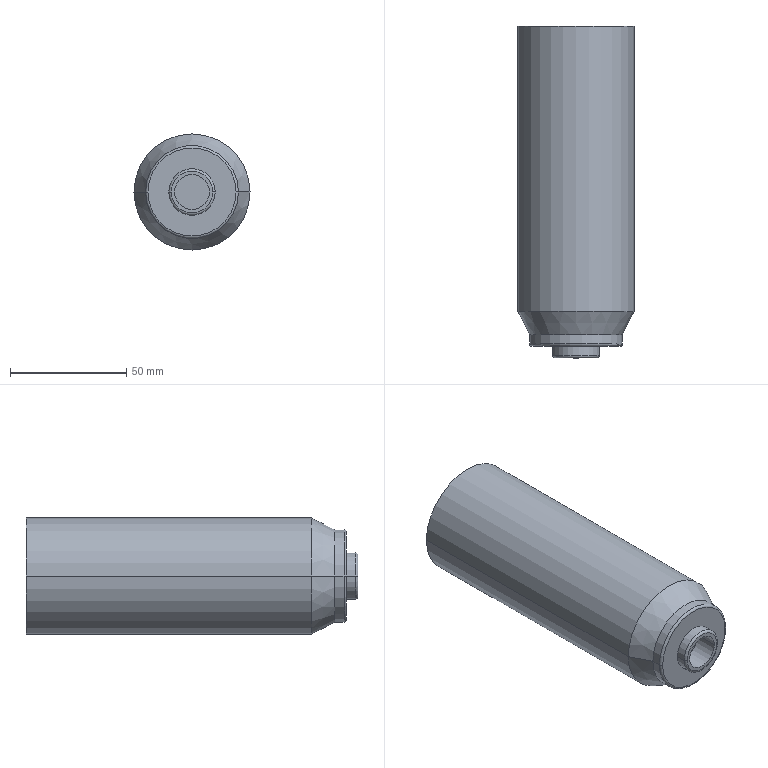Component | SolidWorks | Assembly4.1-1_Ultrasonic.1-1 | 1 solid | 18 faces | box 50 x 143 x 50 mm | volume 263527 mm3 | cylinder 8 | torus 4 | plane 4 | cone 2 | commonest cylinder face diameters 50 x2 40 x2 20 x2 15 x2
build123d program:
from build123d import *


with BuildPart() as part:
    # Sketch1 → Revolve1 (revolve)
    with BuildSketch(Plane.XY, mode=Mode.PRIVATE) as revolve1_sk:
        with BuildLine():
            Line((123, 25), (133, 20))
            Line((133, 20), (137, 20))
            ThreePointArc((137, 20), (137.707, 19.707), (138, 19))
            Line((138, 19), (138, 10))
            Line((138, 10), (142, 10))
            ThreePointArc((142, 10), (142.707, 9.707), (143, 9))
            Line((143, 9), (143, 7.5))
            Line((143, 7.5), (133, 7.5))
            Line((133, 7.5), (133, 0))
            Line((133, 0), (0, 0))
            Line((0, 0), (0, 25))
            Line((0, 25), (123, 25))
        make_face()
    revolve(revolve1_sk.sketch.rotate(Axis((-91.654, 0, 0), (1, 0, 0)), 90), axis=Axis((-91.654, 0, 0), (1, 0, 0)))


solid = part.part

# Placed as in the assembly
solid = solid.moved(Location((0, -101.5, -0.4), (0, 0, -90)))
STEP:
#1=COLOUR_RGB('',0.7922,0.8196,0.9333);
#2=FILL_AREA_STYLE_COLOUR('',#1);
#3=FILL_AREA_STYLE('',(#2));
#4=SURFACE_STYLE_FILL_AREA(#3);
#5=SURFACE_SIDE_STYLE('',(#4));
#6=SURFACE_STYLE_USAGE(.BOTH.,#5);
#7=PRESENTATION_STYLE_ASSIGNMENT((#6));
#8=CARTESIAN_POINT('',(-0.9843,-8.839,-0.01575));
#9=VERTEX_POINT('',#8);
#10=CARTESIAN_POINT('',(0.9843,-8.839,-0.01575));
#11=VERTEX_POINT('',#10);
#12=CARTESIAN_POINT('',(-0.,-8.839,-0.01575));
#13=DIRECTION('',(0.,1.,-0.));
#14=DIRECTION('',(-1.,0.,-0.));
#15=AXIS2_PLACEMENT_3D('',#12,#13,#14);
#16=CIRCLE('',#15,0.9843);
#17=EDGE_CURVE('',#9,#11,#16,.T.);
#18=ORIENTED_EDGE('',*,*,#17,.T.);
#19=CARTESIAN_POINT('',(0.9843,-3.996,-0.01575));
#20=VERTEX_POINT('',#19);
#21=CARTESIAN_POINT('',(0.9843,-0.3877,-0.01575));
#22=DIRECTION('',(0.,1.,-0.));
#23=VECTOR('',#22,39.37);
#24=LINE('',#21,#23);
#25=EDGE_CURVE('',#11,#20,#24,.T.);
#26=ORIENTED_EDGE('',*,*,#25,.T.);
#27=CARTESIAN_POINT('',(-0.9843,-3.996,-0.01575));
#28=VERTEX_POINT('',#27);
#29=CARTESIAN_POINT('',(-0.,-3.996,-0.01575));
#30=DIRECTION('',(0.,1.,-0.));
#31=DIRECTION('',(-1.,0.,-0.));
#32=AXIS2_PLACEMENT_3D('',#29,#30,#31);
#33=CIRCLE('',#32,0.9843);
#34=EDGE_CURVE('',#28,#20,#33,.T.);
#35=ORIENTED_EDGE('',*,*,#34,.F.);
#36=CARTESIAN_POINT('',(-0.9843,-0.3877,-0.01575));
#37=DIRECTION('',(0.,1.,-0.));
#38=VECTOR('',#37,39.37);
#39=LINE('',#36,#38);
#40=EDGE_CURVE('',#9,#28,#39,.T.);
#41=ORIENTED_EDGE('',*,*,#40,.F.);
#42=EDGE_LOOP('',(#18,#26,#35,#41));
#43=FACE_OUTER_BOUND('',#42,.T.);
#44=CARTESIAN_POINT('',(-0.,-0.3877,-0.01575));
#45=DIRECTION('',(0.,1.,-0.));
#46=DIRECTION('',(-1.,0.,-0.));
#47=AXIS2_PLACEMENT_3D('',#44,#45,#46);
#48=CYLINDRICAL_SURFACE('',#47,0.9843);
#49=ADVANCED_FACE('',(#43),#48,.T.);
#50=CARTESIAN_POINT('',(-0.7874,-9.232,-0.01575));
#51=VERTEX_POINT('',#50);
#52=CARTESIAN_POINT('',(0.7874,-9.232,-0.01575));
#53=VERTEX_POINT('',#52);
#54=CARTESIAN_POINT('',(-0.,-9.232,-0.01575));
#55=DIRECTION('',(0.,1.,-0.));
#56=DIRECTION('',(-1.,0.,-0.));
#57=AXIS2_PLACEMENT_3D('',#54,#55,#56);
#58=CIRCLE('',#57,0.7874);
#59=EDGE_CURVE('',#51,#53,#58,.T.);
#60=ORIENTED_EDGE('',*,*,#59,.T.);
#61=CARTESIAN_POINT('',(0.7874,-9.232,-0.01575));
#62=DIRECTION('',(0.4472,0.8944,0.));
#63=VECTOR('',#62,39.37);
#64=LINE('',#61,#63);
#65=EDGE_CURVE('',#53,#11,#64,.T.);
#66=ORIENTED_EDGE('',*,*,#65,.T.);
#67=ORIENTED_EDGE('',*,*,#17,.F.);
#68=CARTESIAN_POINT('',(-0.7874,-9.232,-0.01575));
#69=DIRECTION('',(-0.4472,0.8944,-0.));
#70=VECTOR('',#69,39.37);
#71=LINE('',#68,#70);
#72=EDGE_CURVE('',#51,#9,#71,.T.);
#73=ORIENTED_EDGE('',*,*,#72,.F.);
#74=EDGE_LOOP('',(#60,#66,#67,#73));
#75=FACE_OUTER_BOUND('',#74,.T.);
#76=CARTESIAN_POINT('',(-0.,-9.232,-0.01575));
#77=DIRECTION('',(0.,1.,-0.));
#78=DIRECTION('',(-1.,0.,-0.));
#79=AXIS2_PLACEMENT_3D('',#76,#77,#78);
#80=CONICAL_SURFACE('',#79,0.7874,0.4636);
#81=ADVANCED_FACE('',(#75),#80,.T.);
#82=CARTESIAN_POINT('',(-0.7874,-9.39,-0.01575));
#83=VERTEX_POINT('',#82);
#84=CARTESIAN_POINT('',(0.7874,-9.39,-0.01575));
#85=VERTEX_POINT('',#84);
#86=CARTESIAN_POINT('',(-0.,-9.39,-0.01575));
#87=DIRECTION('',(0.,1.,-0.));
#88=DIRECTION('',(-1.,0.,-0.));
#89=AXIS2_PLACEMENT_3D('',#86,#87,#88);
#90=CIRCLE('',#89,0.7874);
#91=EDGE_CURVE('',#83,#85,#90,.T.);
#92=ORIENTED_EDGE('',*,*,#91,.T.);
#93=CARTESIAN_POINT('',(0.7874,-0.3877,-0.01575));
#94=DIRECTION('',(0.,1.,-0.));
#95=VECTOR('',#94,39.37);
#96=LINE('',#93,#95);
#97=EDGE_CURVE('',#85,#53,#96,.T.);
#98=ORIENTED_EDGE('',*,*,#97,.T.);
#99=ORIENTED_EDGE('',*,*,#59,.F.);
#100=CARTESIAN_POINT('',(-0.7874,-0.3877,-0.01575));
#101=DIRECTION('',(0.,1.,-0.));
#102=VECTOR('',#101,39.37);
#103=LINE('',#100,#102);
#104=EDGE_CURVE('',#83,#51,#103,.T.);
#105=ORIENTED_EDGE('',*,*,#104,.F.);
#106=EDGE_LOOP('',(#92,#98,#99,#105));
#107=FACE_OUTER_BOUND('',#106,.T.);
#108=CARTESIAN_POINT('',(-0.,-0.3877,-0.01575));
#109=DIRECTION('',(0.,1.,-0.));
#110=DIRECTION('',(-1.,0.,-0.));
#111=AXIS2_PLACEMENT_3D('',#108,#109,#110);
#112=CYLINDRICAL_SURFACE('',#111,0.7874);
#113=ADVANCED_FACE('',(#107),#112,.T.);
#114=CARTESIAN_POINT('',(-0.748,-9.429,-0.01575));
#115=VERTEX_POINT('',#114);
#116=CARTESIAN_POINT('',(0.748,-9.429,-0.01575));
#117=VERTEX_POINT('',#116);
#118=CARTESIAN_POINT('',(-0.,-9.429,-0.01575));
#119=DIRECTION('',(0.,1.,-0.));
#120=DIRECTION('',(-1.,0.,-0.));
#121=AXIS2_PLACEMENT_3D('',#118,#119,#120);
#122=CIRCLE('',#121,0.748);
#123=EDGE_CURVE('',#115,#117,#122,.T.);
#124=ORIENTED_EDGE('',*,*,#123,.T.);
#125=CARTESIAN_POINT('',(0.748,-9.39,-0.01575));
#126=DIRECTION('',(-0.,0.,1.));
#127=DIRECTION('',(1.,0.,0.));
#128=AXIS2_PLACEMENT_3D('',#125,#126,#127);
#129=CIRCLE('',#128,0.03937);
#130=EDGE_CURVE('',#117,#85,#129,.T.);
#131=ORIENTED_EDGE('',*,*,#130,.T.);
#132=ORIENTED_EDGE('',*,*,#91,.F.);
#133=CARTESIAN_POINT('',(-0.748,-9.39,-0.01575));
#134=DIRECTION('',(0.,-0.,-1.));
#135=DIRECTION('',(-1.,0.,-0.));
#136=AXIS2_PLACEMENT_3D('',#133,#134,#135);
#137=CIRCLE('',#136,0.03937);
#138=EDGE_CURVE('',#115,#83,#137,.T.);
#139=ORIENTED_EDGE('',*,*,#138,.F.);
#140=EDGE_LOOP('',(#124,#131,#132,#139));
#141=FACE_OUTER_BOUND('',#140,.T.);
#142=CARTESIAN_POINT('',(-0.,-9.39,-0.01575));
#143=DIRECTION('',(0.,1.,-0.));
#144=DIRECTION('',(-1.,0.,-0.));
#145=AXIS2_PLACEMENT_3D('',#142,#143,#144);
#146=TOROIDAL_SURFACE('',#145,0.748,0.03937);
#147=ADVANCED_FACE('',(#141),#146,.T.);
#148=CARTESIAN_POINT('',(-0.3937,-9.587,-0.01575));
#149=VERTEX_POINT('',#148);
#150=CARTESIAN_POINT('',(0.3937,-9.587,-0.01575));
#151=VERTEX_POINT('',#150);
#152=CARTESIAN_POINT('',(-0.,-9.587,-0.01575));
#153=DIRECTION('',(0.,1.,-0.));
#154=DIRECTION('',(-1.,0.,-0.));
#155=AXIS2_PLACEMENT_3D('',#152,#153,#154);
#156=CIRCLE('',#155,0.3937);
#157=EDGE_CURVE('',#149,#151,#156,.T.);
#158=ORIENTED_EDGE('',*,*,#157,.T.);
#159=CARTESIAN_POINT('',(0.3937,-9.429,-0.01575));
#160=VERTEX_POINT('',#159);
#161=CARTESIAN_POINT('',(0.3937,-0.3877,-0.01575));
#162=DIRECTION('',(0.,1.,-0.));
#163=VECTOR('',#162,39.37);
#164=LINE('',#161,#163);
#165=EDGE_CURVE('',#151,#160,#164,.T.);
#166=ORIENTED_EDGE('',*,*,#165,.T.);
#167=CARTESIAN_POINT('',(-0.3937,-9.429,-0.01575));
#168=VERTEX_POINT('',#167);
#169=CARTESIAN_POINT('',(-0.,-9.429,-0.01575));
#170=DIRECTION('',(0.,1.,-0.));
#171=DIRECTION('',(-1.,0.,-0.));
#172=AXIS2_PLACEMENT_3D('',#169,#170,#171);
#173=CIRCLE('',#172,0.3937);
#174=EDGE_CURVE('',#168,#160,#173,.T.);
#175=ORIENTED_EDGE('',*,*,#174,.F.);
#176=CARTESIAN_POINT('',(-0.3937,-0.3877,-0.01575));
#177=DIRECTION('',(0.,1.,-0.));
#178=VECTOR('',#177,39.37);
#179=LINE('',#176,#178);
#180=EDGE_CURVE('',#149,#168,#179,.T.);
#181=ORIENTED_EDGE('',*,*,#180,.F.);
#182=EDGE_LOOP('',(#158,#166,#175,#181));
#183=FACE_OUTER_BOUND('',#182,.T.);
#184=CARTESIAN_POINT('',(-0.,-0.3877,-0.01575));
#185=DIRECTION('',(0.,1.,-0.));
#186=DIRECTION('',(-1.,0.,-0.));
#187=AXIS2_PLACEMENT_3D('',#184,#185,#186);
#188=CYLINDRICAL_SURFACE('',#187,0.3937);
#189=ADVANCED_FACE('',(#183),#188,.T.);
#190=CARTESIAN_POINT('',(-0.3543,-9.626,-0.01575));
#191=VERTEX_POINT('',#190);
#192=CARTESIAN_POINT('',(0.3543,-9.626,-0.01575));
#193=VERTEX_POINT('',#192);
#194=CARTESIAN_POINT('',(-0.,-9.626,-0.01575));
#195=DIRECTION('',(0.,1.,-0.));
#196=DIRECTION('',(-1.,0.,-0.));
#197=AXIS2_PLACEMENT_3D('',#194,#195,#196);
#198=CIRCLE('',#197,0.3543);
#199=EDGE_CURVE('',#191,#193,#198,.T.);
#200=ORIENTED_EDGE('',*,*,#199,.T.);
#201=CARTESIAN_POINT('',(0.3543,-9.587,-0.01575));
#202=DIRECTION('',(-0.,0.,1.));
#203=DIRECTION('',(1.,0.,0.));
#204=AXIS2_PLACEMENT_3D('',#201,#202,#203);
#205=CIRCLE('',#204,0.03937);
#206=EDGE_CURVE('',#193,#151,#205,.T.);
#207=ORIENTED_EDGE('',*,*,#206,.T.);
#208=ORIENTED_EDGE('',*,*,#157,.F.);
#209=CARTESIAN_POINT('',(-0.3543,-9.587,-0.01575));
#210=DIRECTION('',(0.,-0.,-1.));
#211=DIRECTION('',(-1.,0.,-0.));
#212=AXIS2_PLACEMENT_3D('',#209,#210,#211);
#213=CIRCLE('',#212,0.03937);
#214=EDGE_CURVE('',#191,#149,#213,.T.);
#215=ORIENTED_EDGE('',*,*,#214,.F.);
#216=EDGE_LOOP('',(#200,#207,#208,#215));
#217=FACE_OUTER_BOUND('',#216,.T.);
#218=CARTESIAN_POINT('',(-0.,-9.587,-0.01575));
#219=DIRECTION('',(0.,1.,-0.));
#220=DIRECTION('',(-1.,0.,-0.));
#221=AXIS2_PLACEMENT_3D('',#218,#219,#220);
#222=TOROIDAL_SURFACE('',#221,0.3543,0.03937);
#223=ADVANCED_FACE('',(#217),#222,.T.);
#224=CARTESIAN_POINT('',(0.2953,-9.626,-0.01575));
#225=VERTEX_POINT('',#224);
#226=CARTESIAN_POINT('',(-0.2953,-9.626,-0.01575));
#227=VERTEX_POINT('',#226);
#228=CARTESIAN_POINT('',(-0.,-9.626,-0.01575));
#229=DIRECTION('',(0.,1.,-0.));
#230=DIRECTION('',(-1.,0.,-0.));
#231=AXIS2_PLACEMENT_3D('',#228,#229,#230);
#232=CIRCLE('',#231,0.2953);
#233=EDGE_CURVE('',#225,#227,#232,.T.);
#234=ORIENTED_EDGE('',*,*,#233,.F.);
#235=CARTESIAN_POINT('',(0.2953,-9.232,-0.01575));
#236=VERTEX_POINT('',#235);
#237=CARTESIAN_POINT('',(0.2953,-0.3877,-0.01575));
#238=DIRECTION('',(0.,1.,-0.));
#239=VECTOR('',#238,39.37);
#240=LINE('',#237,#239);
#241=EDGE_CURVE('',#225,#236,#240,.T.);
#242=ORIENTED_EDGE('',*,*,#241,.T.);
#243=CARTESIAN_POINT('',(-0.2953,-9.232,-0.01575));
#244=VERTEX_POINT('',#243);
#245=CARTESIAN_POINT('',(-0.,-9.232,-0.01575));
#246=DIRECTION('',(0.,1.,-0.));
#247=DIRECTION('',(-1.,0.,-0.));
#248=AXIS2_PLACEMENT_3D('',#245,#246,#247);
#249=CIRCLE('',#248,0.2953);
#250=EDGE_CURVE('',#236,#244,#249,.T.);
#251=ORIENTED_EDGE('',*,*,#250,.T.);
#252=CARTESIAN_POINT('',(-0.2953,-0.3877,-0.01575));
#253=DIRECTION('',(0.,1.,-0.));
#254=VECTOR('',#253,39.37);
#255=LINE('',#252,#254);
#256=EDGE_CURVE('',#227,#244,#255,.T.);
#257=ORIENTED_EDGE('',*,*,#256,.F.);
#258=EDGE_LOOP('',(#234,#242,#251,#257));
#259=FACE_OUTER_BOUND('',#258,.T.);
#260=CARTESIAN_POINT('',(-0.,-0.3877,-0.01575));
#261=DIRECTION('',(0.,1.,-0.));
#262=DIRECTION('',(-1.,0.,-0.));
#263=AXIS2_PLACEMENT_3D('',#260,#261,#262);
#264=CYLINDRICAL_SURFACE('',#263,0.2953);
#265=ADVANCED_FACE('',(#259),#264,.F.);
#266=ORIENTED_EDGE('',*,*,#34,.T.);
#267=CARTESIAN_POINT('',(-0.,-3.996,-0.01575));
#268=DIRECTION('',(0.,1.,-0.));
#269=DIRECTION('',(-1.,0.,-0.));
#270=AXIS2_PLACEMENT_3D('',#267,#268,#269);
#271=CIRCLE('',#270,0.9843);
#272=EDGE_CURVE('',#20,#28,#271,.T.);
#273=ORIENTED_EDGE('',*,*,#272,.T.);
#274=EDGE_LOOP('',(#266,#273));
#275=FACE_OUTER_BOUND('',#274,.T.);
#276=CARTESIAN_POINT('',(-0.,-3.996,-0.01575));
#277=DIRECTION('',(-0.,-1.,0.));
#278=DIRECTION('',(1.,-0.,0.));
#279=AXIS2_PLACEMENT_3D('',#276,#277,#278);
#280=PLANE('',#279);
#281=ADVANCED_FACE('',(#275),#280,.F.);
#282=CARTESIAN_POINT('',(-0.,-9.232,-0.01575));
#283=DIRECTION('',(0.,1.,-0.));
#284=DIRECTION('',(-1.,0.,-0.));
#285=AXIS2_PLACEMENT_3D('',#282,#283,#284);
#286=CIRCLE('',#285,0.2953);
#287=EDGE_CURVE('',#244,#236,#286,.T.);
#288=ORIENTED_EDGE('',*,*,#287,.F.);
#289=ORIENTED_EDGE('',*,*,#250,.F.);
#290=EDGE_LOOP('',(#288,#289));
#291=FACE_OUTER_BOUND('',#290,.T.);
#292=CARTESIAN_POINT('',(-0.,-9.232,-0.311));
#293=DIRECTION('',(0.,1.,-0.));
#294=DIRECTION('',(-1.,0.,-0.));
#295=AXIS2_PLACEMENT_3D('',#292,#293,#294);
#296=PLANE('',#295);
#297=ADVANCED_FACE('',(#291),#296,.F.);
#298=ORIENTED_EDGE('',*,*,#241,.F.);
#299=CARTESIAN_POINT('',(-0.,-9.626,-0.01575));
#300=DIRECTION('',(0.,1.,-0.));
#301=DIRECTION('',(-1.,0.,-0.));
#302=AXIS2_PLACEMENT_3D('',#299,#300,#301);
#303=CIRCLE('',#302,0.2953);
#304=EDGE_CURVE('',#227,#225,#303,.T.);
#305=ORIENTED_EDGE('',*,*,#304,.F.);
#306=ORIENTED_EDGE('',*,*,#256,.T.);
#307=ORIENTED_EDGE('',*,*,#287,.T.);
#308=EDGE_LOOP('',(#298,#305,#306,#307));
#309=FACE_OUTER_BOUND('',#308,.T.);
#310=CARTESIAN_POINT('',(-0.,-0.3877,-0.01575));
#311=DIRECTION('',(0.,1.,-0.));
#312=DIRECTION('',(-1.,0.,-0.));
#313=AXIS2_PLACEMENT_3D('',#310,#311,#312);
#314=CYLINDRICAL_SURFACE('',#313,0.2953);
#315=ADVANCED_FACE('',(#309),#314,.F.);
#316=ORIENTED_EDGE('',*,*,#199,.F.);
#317=CARTESIAN_POINT('',(-0.,-9.626,-0.01575));
#318=DIRECTION('',(0.,1.,-0.));
#319=DIRECTION('',(-1.,0.,-0.));
#320=AXIS2_PLACEMENT_3D('',#317,#318,#319);
#321=CIRCLE('',#320,0.3543);
#322=EDGE_CURVE('',#193,#191,#321,.T.);
#323=ORIENTED_EDGE('',*,*,#322,.F.);
#324=EDGE_LOOP('',(#316,#323));
#325=FACE_OUTER_BOUND('',#324,.T.);
#326=ORIENTED_EDGE('',*,*,#304,.T.);
#327=ORIENTED_EDGE('',*,*,#233,.T.);
#328=EDGE_LOOP('',(#326,#327));
#329=FACE_BOUND('',#328,.T.);
#330=CARTESIAN_POINT('',(-0.,-9.626,-0.3701));
#331=DIRECTION('',(0.,1.,-0.));
#332=DIRECTION('',(-1.,0.,-0.));
#333=AXIS2_PLACEMENT_3D('',#330,#331,#332);
#334=PLANE('',#333);
#335=ADVANCED_FACE('',(#325,#329),#334,.F.);
#336=ORIENTED_EDGE('',*,*,#206,.F.);
#337=ORIENTED_EDGE('',*,*,#322,.T.);
#338=ORIENTED_EDGE('',*,*,#214,.T.);
#339=CARTESIAN_POINT('',(-0.,-9.587,-0.01575));
#340=DIRECTION('',(0.,1.,-0.));
#341=DIRECTION('',(-1.,0.,-0.));
#342=AXIS2_PLACEMENT_3D('',#339,#340,#341);
#343=CIRCLE('',#342,0.3937);
#344=EDGE_CURVE('',#151,#149,#343,.T.);
#345=ORIENTED_EDGE('',*,*,#344,.F.);
#346=EDGE_LOOP('',(#336,#337,#338,#345));
#347=FACE_OUTER_BOUND('',#346,.T.);
#348=CARTESIAN_POINT('',(-0.,-9.587,-0.01575));
#349=DIRECTION('',(0.,1.,-0.));
#350=DIRECTION('',(-1.,0.,-0.));
#351=AXIS2_PLACEMENT_3D('',#348,#349,#350);
#352=TOROIDAL_SURFACE('',#351,0.3543,0.03937);
#353=ADVANCED_FACE('',(#347),#352,.T.);
#354=ORIENTED_EDGE('',*,*,#165,.F.);
#355=ORIENTED_EDGE('',*,*,#344,.T.);
#356=ORIENTED_EDGE('',*,*,#180,.T.);
#357=CARTESIAN_POINT('',(-0.,-9.429,-0.01575));
#358=DIRECTION('',(0.,1.,-0.));
#359=DIRECTION('',(-1.,0.,-0.));
#360=AXIS2_PLACEMENT_3D('',#357,#358,#359);
#361=CIRCLE('',#360,0.3937);
#362=EDGE_CURVE('',#160,#168,#361,.T.);
#363=ORIENTED_EDGE('',*,*,#362,.F.);
#364=EDGE_LOOP('',(#354,#355,#356,#363));
#365=FACE_OUTER_BOUND('',#364,.T.);
#366=CARTESIAN_POINT('',(-0.,-0.3877,-0.01575));
#367=DIRECTION('',(0.,1.,-0.));
#368=DIRECTION('',(-1.,0.,-0.));
#369=AXIS2_PLACEMENT_3D('',#366,#367,#368);
#370=CYLINDRICAL_SURFACE('',#369,0.3937);
#371=ADVANCED_FACE('',(#365),#370,.T.);
#372=ORIENTED_EDGE('',*,*,#123,.F.);
#373=CARTESIAN_POINT('',(-0.,-9.429,-0.01575));
#374=DIRECTION('',(0.,1.,-0.));
#375=DIRECTION('',(-1.,0.,-0.));
#376=AXIS2_PLACEMENT_3D('',#373,#374,#375);
#377=CIRCLE('',#376,0.748);
#378=EDGE_CURVE('',#117,#115,#377,.T.);
#379=ORIENTED_EDGE('',*,*,#378,.F.);
#380=EDGE_LOOP('',(#372,#379));
#381=FACE_OUTER_BOUND('',#380,.T.);
#382=ORIENTED_EDGE('',*,*,#174,.T.);
#383=ORIENTED_EDGE('',*,*,#362,.T.);
#384=EDGE_LOOP('',(#382,#383));
#385=FACE_BOUND('',#384,.T.);
#386=CARTESIAN_POINT('',(-0.,-9.429,-0.7638));
#387=DIRECTION('',(0.,1.,-0.));
#388=DIRECTION('',(-1.,0.,-0.));
#389=AXIS2_PLACEMENT_3D('',#386,#387,#388);
#390=PLANE('',#389);
#391=ADVANCED_FACE('',(#381,#385),#390,.F.);
#392=ORIENTED_EDGE('',*,*,#130,.F.);
#393=ORIENTED_EDGE('',*,*,#378,.T.);
#394=ORIENTED_EDGE('',*,*,#138,.T.);
#395=CARTESIAN_POINT('',(-0.,-9.39,-0.01575));
#396=DIRECTION('',(0.,1.,-0.));
#397=DIRECTION('',(-1.,0.,-0.));
#398=AXIS2_PLACEMENT_3D('',#395,#396,#397);
#399=CIRCLE('',#398,0.7874);
#400=EDGE_CURVE('',#85,#83,#399,.T.);
#401=ORIENTED_EDGE('',*,*,#400,.F.);
#402=EDGE_LOOP('',(#392,#393,#394,#401));
#403=FACE_OUTER_BOUND('',#402,.T.);
#404=CARTESIAN_POINT('',(-0.,-9.39,-0.01575));
#405=DIRECTION('',(0.,1.,-0.));
#406=DIRECTION('',(-1.,0.,-0.));
#407=AXIS2_PLACEMENT_3D('',#404,#405,#406);
#408=TOROIDAL_SURFACE('',#407,0.748,0.03937);
#409=ADVANCED_FACE('',(#403),#408,.T.);
#410=ORIENTED_EDGE('',*,*,#97,.F.);
#411=ORIENTED_EDGE('',*,*,#400,.T.);
#412=ORIENTED_EDGE('',*,*,#104,.T.);
#413=CARTESIAN_POINT('',(-0.,-9.232,-0.01575));
#414=DIRECTION('',(0.,1.,-0.));
#415=DIRECTION('',(-1.,0.,-0.));
#416=AXIS2_PLACEMENT_3D('',#413,#414,#415);
#417=CIRCLE('',#416,0.7874);
#418=EDGE_CURVE('',#53,#51,#417,.T.);
#419=ORIENTED_EDGE('',*,*,#418,.F.);
#420=EDGE_LOOP('',(#410,#411,#412,#419));
#421=FACE_OUTER_BOUND('',#420,.T.);
#422=CARTESIAN_POINT('',(-0.,-0.3877,-0.01575));
#423=DIRECTION('',(0.,1.,-0.));
#424=DIRECTION('',(-1.,0.,-0.));
#425=AXIS2_PLACEMENT_3D('',#422,#423,#424);
#426=CYLINDRICAL_SURFACE('',#425,0.7874);
#427=ADVANCED_FACE('',(#421),#426,.T.);
#428=ORIENTED_EDGE('',*,*,#65,.F.);
#429=ORIENTED_EDGE('',*,*,#418,.T.);
#430=ORIENTED_EDGE('',*,*,#72,.T.);
#431=CARTESIAN_POINT('',(-0.,-8.839,-0.01575));
#432=DIRECTION('',(0.,1.,-0.));
#433=DIRECTION('',(-1.,0.,-0.));
#434=AXIS2_PLACEMENT_3D('',#431,#432,#433);
#435=CIRCLE('',#434,0.9843);
#436=EDGE_CURVE('',#11,#9,#435,.T.);
#437=ORIENTED_EDGE('',*,*,#436,.F.);
#438=EDGE_LOOP('',(#428,#429,#430,#437));
#439=FACE_OUTER_BOUND('',#438,.T.);
#440=CARTESIAN_POINT('',(-0.,-9.232,-0.01575));
#441=DIRECTION('',(0.,1.,-0.));
#442=DIRECTION('',(-1.,0.,-0.));
#443=AXIS2_PLACEMENT_3D('',#440,#441,#442);
#444=CONICAL_SURFACE('',#443,0.7874,0.4636);
#445=ADVANCED_FACE('',(#439),#444,.T.);
#446=ORIENTED_EDGE('',*,*,#25,.F.);
#447=ORIENTED_EDGE('',*,*,#436,.T.);
#448=ORIENTED_EDGE('',*,*,#40,.T.);
#449=ORIENTED_EDGE('',*,*,#272,.F.);
#450=EDGE_LOOP('',(#446,#447,#448,#449));
#451=FACE_OUTER_BOUND('',#450,.T.);
#452=CARTESIAN_POINT('',(-0.,-0.3877,-0.01575));
#453=DIRECTION('',(0.,1.,-0.));
#454=DIRECTION('',(-1.,0.,-0.));
#455=AXIS2_PLACEMENT_3D('',#452,#453,#454);
#456=CYLINDRICAL_SURFACE('',#455,0.9843);
#457=ADVANCED_FACE('',(#451),#456,.T.);
#458=CLOSED_SHELL('',(#49,#81,#113,#147,#189,#223,#265,#281,#297,#315,#335,#353,#371,#391,#409,#427,#445,#457));
#459=MANIFOLD_SOLID_BREP('',#458);
#460=STYLED_ITEM('',(#7),#459);
#461=(LENGTH_UNIT()NAMED_UNIT(*)SI_UNIT($,.METRE.));
#462=LENGTH_MEASURE_WITH_UNIT(LENGTH_MEASURE(0.0254),#461);
#463=DIMENSIONAL_EXPONENTS(1.,0.,0.,0.,0.,0.,0.);
#464=(CONVERSION_BASED_UNIT('',#462)LENGTH_UNIT()NAMED_UNIT(#463));
#465=UNCERTAINTY_MEASURE_WITH_UNIT(LENGTH_MEASURE(0.00001),#464,'','');
#466=(NAMED_UNIT(*)PLANE_ANGLE_UNIT()SI_UNIT($,.RADIAN.));
#467=(NAMED_UNIT(*)SI_UNIT($,.STERADIAN.)SOLID_ANGLE_UNIT());
#468=(GEOMETRIC_REPRESENTATION_CONTEXT(3)GLOBAL_UNCERTAINTY_ASSIGNED_CONTEXT((#465))GLOBAL_UNIT_ASSIGNED_CONTEXT((#464,#466,#467))REPRESENTATION_CONTEXT('',''));
#469=MECHANICAL_DESIGN_GEOMETRIC_PRESENTATION_REPRESENTATION('',(#460),#468);
#470=PRESENTATION_LAYER_ASSIGNMENT('','',(#460));
#471=CARTESIAN_POINT('',(0.,0.,0.));
#472=DIRECTION('',(0.,0.,1.));
#473=DIRECTION('',(1.,0.,0.));
#474=AXIS2_PLACEMENT_3D('',#471,#472,#473);
#475=(LENGTH_UNIT()NAMED_UNIT(*)SI_UNIT($,.METRE.));
#476=LENGTH_MEASURE_WITH_UNIT(LENGTH_MEASURE(0.0254),#475);
#477=DIMENSIONAL_EXPONENTS(1.,0.,0.,0.,0.,0.,0.);
#478=(CONVERSION_BASED_UNIT('',#476)LENGTH_UNIT()NAMED_UNIT(#477));
#479=UNCERTAINTY_MEASURE_WITH_UNIT(LENGTH_MEASURE(0.00001),#478,'','');
#480=(NAMED_UNIT(*)PLANE_ANGLE_UNIT()SI_UNIT($,.RADIAN.));
#481=(NAMED_UNIT(*)SI_UNIT($,.STERADIAN.)SOLID_ANGLE_UNIT());
#482=(GEOMETRIC_REPRESENTATION_CONTEXT(3)GLOBAL_UNCERTAINTY_ASSIGNED_CONTEXT((#479))GLOBAL_UNIT_ASSIGNED_CONTEXT((#478,#480,#481))REPRESENTATION_CONTEXT('',''));
#483=ADVANCED_BREP_SHAPE_REPRESENTATION('',(#459,#474),#482);